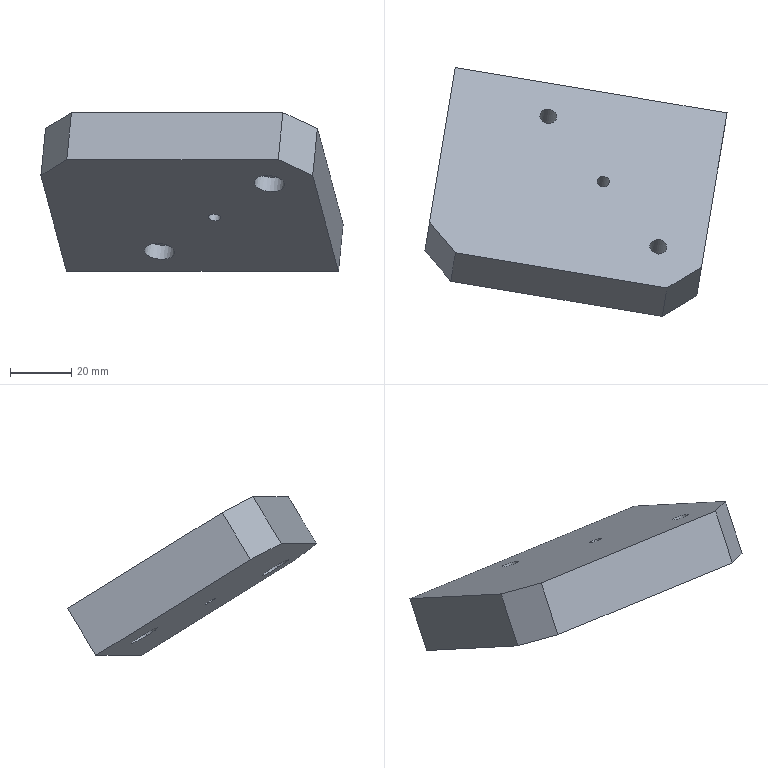Component | SolidWorks | 14AC-24-1-007-1 | 1 solid | 28 faces | box 98.73 x 81.3 x 51.9 mm | volume 109240 mm3 | cylinder 14 | plane 10 | cone 4 | commonest cylinder face diameters 10 x4 5.5 x4 5 x4 4 x2
build123d program:
from build123d import *

# Parameters (mm, degrees)
SKETCH1_W                                       = 90
SKETCH1_H                                       = 70
BOSS_EXTRUDE1_DEPTH                             = 18
CHAMFER1_SIZE                                   = 10
LPATTERN1_COUNT                                 = 2
LPATTERN1_PITCH                                 = 33
M5_HEX_SOCKET_HEAD_CAP_SCREW_CBORE1_D           = 5.5
M5_HEX_SOCKET_HEAD_CAP_SCREW_CBORE1_CBORE_D     = 10
M5_HEX_SOCKET_HEAD_CAP_SCREW_CBORE1_CBORE_DEPTH = 5.4
SKETCH12_R                                      = 2
CUT_EXTRUDE6_DEPTH                              = 116.43


with BuildPart() as part:
    # Sketch1 → Boss-Extrude1 (new body)
    with BuildSketch(Plane.XY):
        with Locations((45, 35)):
            Rectangle(SKETCH1_W, SKETCH1_H)
    extrude(amount=BOSS_EXTRUDE1_DEPTH)

    # Chamfer1
    chamfer1_edges = [part.edges().sort_by_distance(p)[0] for p in [
        (0, 70, 9),
        (90, 70, 9),
    ]]
    chamfer(chamfer1_edges, length=CHAMFER1_SIZE)

    # Sketch8 → M6 Tapped Hole1 (revolve, cut)
    with BuildSketch(Plane(origin=(18, 0, 9), x_dir=(0, 0, -1), z_dir=(1, 0, 0))):
        Polygon((0, 0), (0, 18.502), (2.5, 17), (2.5, 0), align=None)
    m6_tapped_hole1 = revolve(axis=Axis((18, -6.35, 9), (0, 1, 0)), mode=Mode.SUBTRACT)

    # LPattern1: M6 Tapped Hole1 ×2
    with Locations(*[(i * LPATTERN1_PITCH, 0, 0) for i in range(1, LPATTERN1_COUNT)]):
        add(m6_tapped_hole1, mode=Mode.SUBTRACT)

    # M5 Hex Socket Head Cap Screw CBORE1 (through all)
    with Locations(Plane(origin=(15, 55, 0), x_dir=(-1, 0, 0), z_dir=(0, 0, -1))):
        with Locations((0, 0), (-42.426, -42.426)):
            CounterBoreHole(M5_HEX_SOCKET_HEAD_CAP_SCREW_CBORE1_D / 2, M5_HEX_SOCKET_HEAD_CAP_SCREW_CBORE1_CBORE_D / 2, M5_HEX_SOCKET_HEAD_CAP_SCREW_CBORE1_CBORE_DEPTH)

    # Sketch12 → Cut-Extrude6 (cut, through all)
    with BuildSketch(Plane(origin=(0, 0, 0), x_dir=(-1, 0, 0), z_dir=(0, 0, -1))):
        with Locations((-36.213, 33.787)):
            Circle(SKETCH12_R)
    extrude(amount=-CUT_EXTRUDE6_DEPTH, mode=Mode.SUBTRACT)


solid = part.part

# Placed as in the assembly
solid = solid.moved(Location((507.217, -245.357, -123.864), (-31.129, 4.92, 171.918)))
STEP:
#1=CARTESIAN_POINT('',(18.36,-10.167,-3.578));
#2=VERTEX_POINT('',#1);
#3=CARTESIAN_POINT('',(18.515,-10.193,-3.578));
#4=VERTEX_POINT('',#3);
#5=CARTESIAN_POINT('',(18.437,-10.18,-3.578));
#6=DIRECTION('',(-0.08576,-0.5151,-0.8529));
#7=DIRECTION('',(0.9864,-0.1642,0.));
#8=AXIS2_PLACEMENT_3D('',#5,#6,#7);
#9=CIRCLE('',#8,0.07874);
#10=EDGE_CURVE('',#2,#4,#9,.T.);
#11=ORIENTED_EDGE('',*,*,#10,.F.);
#12=CARTESIAN_POINT('',(18.299,-10.532,-4.182));
#13=VERTEX_POINT('',#12);
#14=CARTESIAN_POINT('',(18.36,-10.167,-3.578));
#15=DIRECTION('',(-0.08576,-0.5151,-0.8529));
#16=VECTOR('',#15,39.37);
#17=LINE('',#14,#16);
#18=EDGE_CURVE('',#2,#13,#17,.T.);
#19=ORIENTED_EDGE('',*,*,#18,.T.);
#20=CARTESIAN_POINT('',(18.454,-10.558,-4.182));
#21=VERTEX_POINT('',#20);
#22=CARTESIAN_POINT('',(18.376,-10.545,-4.182));
#23=DIRECTION('',(-0.08576,-0.5151,-0.8529));
#24=DIRECTION('',(0.9864,-0.1642,0.));
#25=AXIS2_PLACEMENT_3D('',#22,#23,#24);
#26=CIRCLE('',#25,0.07874);
#27=EDGE_CURVE('',#13,#21,#26,.T.);
#28=ORIENTED_EDGE('',*,*,#27,.T.);
#29=CARTESIAN_POINT('',(18.515,-10.193,-3.578));
#30=DIRECTION('',(-0.08576,-0.5151,-0.8529));
#31=VECTOR('',#30,39.37);
#32=LINE('',#29,#31);
#33=EDGE_CURVE('',#4,#21,#32,.T.);
#34=ORIENTED_EDGE('',*,*,#33,.F.);
#35=EDGE_LOOP('',(#11,#19,#28,#34));
#36=FACE_OUTER_BOUND('',#35,.T.);
#37=CARTESIAN_POINT('',(18.437,-10.18,-3.578));
#38=DIRECTION('',(-0.08576,-0.5151,-0.8529));
#39=DIRECTION('',(0.9864,-0.1642,0.));
#40=AXIS2_PLACEMENT_3D('',#37,#38,#39);
#41=CYLINDRICAL_SURFACE('',#40,0.07874);
#42=ADVANCED_FACE('',(#36),#41,.F.);
#43=CARTESIAN_POINT('',(18.907,-11.243,-3.565));
#44=VERTEX_POINT('',#43);
#45=CARTESIAN_POINT('',(19.296,-11.307,-3.565));
#46=VERTEX_POINT('',#45);
#47=CARTESIAN_POINT('',(19.102,-11.275,-3.565));
#48=DIRECTION('',(-0.08576,-0.5151,-0.8529));
#49=DIRECTION('',(0.9864,-0.1642,0.));
#50=AXIS2_PLACEMENT_3D('',#47,#48,#49);
#51=CIRCLE('',#50,0.1969);
#52=EDGE_CURVE('',#44,#46,#51,.T.);
#53=ORIENTED_EDGE('',*,*,#52,.F.);
#54=CARTESIAN_POINT('',(18.889,-11.352,-3.746));
#55=VERTEX_POINT('',#54);
#56=CARTESIAN_POINT('',(18.889,-11.352,-3.746));
#57=DIRECTION('',(-0.08576,-0.5151,-0.8529));
#58=VECTOR('',#57,39.37);
#59=LINE('',#56,#58);
#60=EDGE_CURVE('',#44,#55,#59,.T.);
#61=ORIENTED_EDGE('',*,*,#60,.T.);
#62=CARTESIAN_POINT('',(19.277,-11.417,-3.746));
#63=VERTEX_POINT('',#62);
#64=CARTESIAN_POINT('',(19.083,-11.384,-3.746));
#65=DIRECTION('',(-0.08576,-0.5151,-0.8529));
#66=DIRECTION('',(0.9864,-0.1642,0.));
#67=AXIS2_PLACEMENT_3D('',#64,#65,#66);
#68=CIRCLE('',#67,0.1969);
#69=EDGE_CURVE('',#55,#63,#68,.T.);
#70=ORIENTED_EDGE('',*,*,#69,.T.);
#71=CARTESIAN_POINT('',(19.277,-11.417,-3.746));
#72=DIRECTION('',(-0.08576,-0.5151,-0.8529));
#73=VECTOR('',#72,39.37);
#74=LINE('',#71,#73);
#75=EDGE_CURVE('',#46,#63,#74,.T.);
#76=ORIENTED_EDGE('',*,*,#75,.F.);
#77=EDGE_LOOP('',(#53,#61,#70,#76));
#78=FACE_OUTER_BOUND('',#77,.T.);
#79=CARTESIAN_POINT('',(19.083,-11.384,-3.746));
#80=DIRECTION('',(-0.08576,-0.5151,-0.8529));
#81=DIRECTION('',(0.9864,-0.1642,0.));
#82=AXIS2_PLACEMENT_3D('',#79,#80,#81);
#83=CYLINDRICAL_SURFACE('',#82,0.1969);
#84=ADVANCED_FACE('',(#78),#83,.F.);
#85=CARTESIAN_POINT('',(19.037,-11.002,-3.142));
#86=VERTEX_POINT('',#85);
#87=CARTESIAN_POINT('',(19.251,-11.037,-3.142));
#88=VERTEX_POINT('',#87);
#89=CARTESIAN_POINT('',(19.144,-11.019,-3.142));
#90=DIRECTION('',(-0.08576,-0.5151,-0.8529));
#91=DIRECTION('',(0.9864,-0.1642,0.));
#92=AXIS2_PLACEMENT_3D('',#89,#90,#91);
#93=CIRCLE('',#92,0.1083);
#94=EDGE_CURVE('',#86,#88,#93,.T.);
#95=ORIENTED_EDGE('',*,*,#94,.F.);
#96=CARTESIAN_POINT('',(18.995,-11.257,-3.565));
#97=VERTEX_POINT('',#96);
#98=CARTESIAN_POINT('',(18.977,-11.367,-3.746));
#99=DIRECTION('',(-0.08576,-0.5151,-0.8529));
#100=VECTOR('',#99,39.37);
#101=LINE('',#98,#100);
#102=EDGE_CURVE('',#86,#97,#101,.T.);
#103=ORIENTED_EDGE('',*,*,#102,.T.);
#104=CARTESIAN_POINT('',(19.208,-11.293,-3.565));
#105=VERTEX_POINT('',#104);
#106=CARTESIAN_POINT('',(19.102,-11.275,-3.565));
#107=DIRECTION('',(-0.08576,-0.5151,-0.8529));
#108=DIRECTION('',(0.9864,-0.1642,0.));
#109=AXIS2_PLACEMENT_3D('',#106,#107,#108);
#110=CIRCLE('',#109,0.1083);
#111=EDGE_CURVE('',#97,#105,#110,.T.);
#112=ORIENTED_EDGE('',*,*,#111,.T.);
#113=CARTESIAN_POINT('',(19.19,-11.402,-3.746));
#114=DIRECTION('',(-0.08576,-0.5151,-0.8529));
#115=VECTOR('',#114,39.37);
#116=LINE('',#113,#115);
#117=EDGE_CURVE('',#88,#105,#116,.T.);
#118=ORIENTED_EDGE('',*,*,#117,.F.);
#119=EDGE_LOOP('',(#95,#103,#112,#118));
#120=FACE_OUTER_BOUND('',#119,.T.);
#121=CARTESIAN_POINT('',(19.083,-11.384,-3.746));
#122=DIRECTION('',(-0.08576,-0.5151,-0.8529));
#123=DIRECTION('',(0.9864,-0.1642,0.));
#124=AXIS2_PLACEMENT_3D('',#121,#122,#123);
#125=CYLINDRICAL_SURFACE('',#124,0.1083);
#126=ADVANCED_FACE('',(#120),#125,.F.);
#127=CARTESIAN_POINT('',(17.494,-9.563,-4.437));
#128=VERTEX_POINT('',#127);
#129=CARTESIAN_POINT('',(17.882,-9.628,-4.437));
#130=VERTEX_POINT('',#129);
#131=CARTESIAN_POINT('',(17.688,-9.595,-4.437));
#132=DIRECTION('',(-0.08576,-0.5151,-0.8529));
#133=DIRECTION('',(0.9864,-0.1642,0.));
#134=AXIS2_PLACEMENT_3D('',#131,#132,#133);
#135=CIRCLE('',#134,0.1969);
#136=EDGE_CURVE('',#128,#130,#135,.T.);
#137=ORIENTED_EDGE('',*,*,#136,.F.);
#138=CARTESIAN_POINT('',(17.475,-9.673,-4.618));
#139=VERTEX_POINT('',#138);
#140=CARTESIAN_POINT('',(17.475,-9.673,-4.618));
#141=DIRECTION('',(-0.08576,-0.5151,-0.8529));
#142=VECTOR('',#141,39.37);
#143=LINE('',#140,#142);
#144=EDGE_CURVE('',#128,#139,#143,.T.);
#145=ORIENTED_EDGE('',*,*,#144,.T.);
#146=CARTESIAN_POINT('',(17.864,-9.737,-4.618));
#147=VERTEX_POINT('',#146);
#148=CARTESIAN_POINT('',(17.67,-9.705,-4.618));
#149=DIRECTION('',(-0.08576,-0.5151,-0.8529));
#150=DIRECTION('',(0.9864,-0.1642,0.));
#151=AXIS2_PLACEMENT_3D('',#148,#149,#150);
#152=CIRCLE('',#151,0.1969);
#153=EDGE_CURVE('',#139,#147,#152,.T.);
#154=ORIENTED_EDGE('',*,*,#153,.T.);
#155=CARTESIAN_POINT('',(17.864,-9.737,-4.618));
#156=DIRECTION('',(-0.08576,-0.5151,-0.8529));
#157=VECTOR('',#156,39.37);
#158=LINE('',#155,#157);
#159=EDGE_CURVE('',#130,#147,#158,.T.);
#160=ORIENTED_EDGE('',*,*,#159,.F.);
#161=EDGE_LOOP('',(#137,#145,#154,#160));
#162=FACE_OUTER_BOUND('',#161,.T.);
#163=CARTESIAN_POINT('',(17.67,-9.705,-4.618));
#164=DIRECTION('',(-0.08576,-0.5151,-0.8529));
#165=DIRECTION('',(0.9864,-0.1642,0.));
#166=AXIS2_PLACEMENT_3D('',#163,#164,#165);
#167=CYLINDRICAL_SURFACE('',#166,0.1969);
#168=ADVANCED_FACE('',(#162),#167,.F.);
#169=CARTESIAN_POINT('',(17.624,-9.322,-4.014));
#170=VERTEX_POINT('',#169);
#171=CARTESIAN_POINT('',(17.837,-9.358,-4.014));
#172=VERTEX_POINT('',#171);
#173=CARTESIAN_POINT('',(17.73,-9.34,-4.014));
#174=DIRECTION('',(-0.08576,-0.5151,-0.8529));
#175=DIRECTION('',(0.9864,-0.1642,0.));
#176=AXIS2_PLACEMENT_3D('',#173,#174,#175);
#177=CIRCLE('',#176,0.1083);
#178=EDGE_CURVE('',#170,#172,#177,.T.);
#179=ORIENTED_EDGE('',*,*,#178,.F.);
#180=CARTESIAN_POINT('',(17.581,-9.578,-4.437));
#181=VERTEX_POINT('',#180);
#182=CARTESIAN_POINT('',(17.563,-9.687,-4.618));
#183=DIRECTION('',(-0.08576,-0.5151,-0.8529));
#184=VECTOR('',#183,39.37);
#185=LINE('',#182,#184);
#186=EDGE_CURVE('',#170,#181,#185,.T.);
#187=ORIENTED_EDGE('',*,*,#186,.T.);
#188=CARTESIAN_POINT('',(17.795,-9.613,-4.437));
#189=VERTEX_POINT('',#188);
#190=CARTESIAN_POINT('',(17.688,-9.595,-4.437));
#191=DIRECTION('',(-0.08576,-0.5151,-0.8529));
#192=DIRECTION('',(0.9864,-0.1642,0.));
#193=AXIS2_PLACEMENT_3D('',#190,#191,#192);
#194=CIRCLE('',#193,0.1083);
#195=EDGE_CURVE('',#181,#189,#194,.T.);
#196=ORIENTED_EDGE('',*,*,#195,.T.);
#197=CARTESIAN_POINT('',(17.776,-9.723,-4.618));
#198=DIRECTION('',(-0.08576,-0.5151,-0.8529));
#199=VECTOR('',#198,39.37);
#200=LINE('',#197,#199);
#201=EDGE_CURVE('',#172,#189,#200,.T.);
#202=ORIENTED_EDGE('',*,*,#201,.F.);
#203=EDGE_LOOP('',(#179,#187,#196,#202));
#204=FACE_OUTER_BOUND('',#203,.T.);
#205=CARTESIAN_POINT('',(17.67,-9.705,-4.618));
#206=DIRECTION('',(-0.08576,-0.5151,-0.8529));
#207=DIRECTION('',(0.9864,-0.1642,0.));
#208=AXIS2_PLACEMENT_3D('',#205,#206,#207);
#209=CYLINDRICAL_SURFACE('',#208,0.1083);
#210=ADVANCED_FACE('',(#204),#209,.F.);
#211=CARTESIAN_POINT('',(17.934,-9.66,-4.141));
#212=VERTEX_POINT('',#211);
#213=CARTESIAN_POINT('',(17.917,-9.761,-4.309));
#214=VERTEX_POINT('',#213);
#215=CARTESIAN_POINT('',(17.925,-9.711,-4.225));
#216=DIRECTION('',(0.1401,0.8413,-0.5222));
#217=DIRECTION('',(-0.08576,-0.5151,-0.8529));
#218=AXIS2_PLACEMENT_3D('',#215,#216,#217);
#219=CIRCLE('',#218,0.09843);
#220=EDGE_CURVE('',#212,#214,#219,.T.);
#221=ORIENTED_EDGE('',*,*,#220,.F.);
#222=CARTESIAN_POINT('',(18.027,-9.097,-4.49));
#223=VERTEX_POINT('',#222);
#224=CARTESIAN_POINT('',(18.027,-9.097,-4.49));
#225=DIRECTION('',(0.1401,0.8413,-0.5222));
#226=VECTOR('',#225,39.37);
#227=LINE('',#224,#226);
#228=EDGE_CURVE('',#212,#223,#227,.T.);
#229=ORIENTED_EDGE('',*,*,#228,.T.);
#230=CARTESIAN_POINT('',(18.01,-9.198,-4.658));
#231=VERTEX_POINT('',#230);
#232=CARTESIAN_POINT('',(18.019,-9.147,-4.574));
#233=DIRECTION('',(0.1401,0.8413,-0.5222));
#234=DIRECTION('',(-0.08576,-0.5151,-0.8529));
#235=AXIS2_PLACEMENT_3D('',#232,#233,#234);
#236=CIRCLE('',#235,0.09843);
#237=EDGE_CURVE('',#223,#231,#236,.T.);
#238=ORIENTED_EDGE('',*,*,#237,.T.);
#239=CARTESIAN_POINT('',(18.01,-9.198,-4.658));
#240=DIRECTION('',(0.1401,0.8413,-0.5222));
#241=VECTOR('',#240,39.37);
#242=LINE('',#239,#241);
#243=EDGE_CURVE('',#214,#231,#242,.T.);
#244=ORIENTED_EDGE('',*,*,#243,.F.);
#245=EDGE_LOOP('',(#221,#229,#238,#244));
#246=FACE_OUTER_BOUND('',#245,.T.);
#247=CARTESIAN_POINT('',(18.019,-9.147,-4.574));
#248=DIRECTION('',(0.1401,0.8413,-0.5222));
#249=DIRECTION('',(-0.08576,-0.5151,-0.8529));
#250=AXIS2_PLACEMENT_3D('',#247,#248,#249);
#251=CYLINDRICAL_SURFACE('',#250,0.09843);
#252=ADVANCED_FACE('',(#246),#251,.F.);
#253=CARTESIAN_POINT('',(17.917,-9.76,-4.194));
#254=VERTEX_POINT('',#253);
#255=CARTESIAN_POINT('',(17.917,-9.761,-4.309));
#256=DIRECTION('',(-0.001367,-0.008211,-1.));
#257=VECTOR('',#256,39.37);
#258=LINE('',#255,#257);
#259=EDGE_CURVE('',#254,#214,#258,.T.);
#260=ORIENTED_EDGE('',*,*,#259,.F.);
#261=CARTESIAN_POINT('',(17.934,-9.66,-4.141));
#262=DIRECTION('',(0.1457,0.8748,0.4621));
#263=VECTOR('',#262,39.37);
#264=LINE('',#261,#263);
#265=EDGE_CURVE('',#254,#212,#264,.T.);
#266=ORIENTED_EDGE('',*,*,#265,.T.);
#267=ORIENTED_EDGE('',*,*,#220,.T.);
#268=EDGE_LOOP('',(#260,#266,#267));
#269=FACE_OUTER_BOUND('',#268,.T.);
#270=CARTESIAN_POINT('',(17.925,-9.711,-4.225));
#271=DIRECTION('',(0.1401,0.8413,-0.5222));
#272=DIRECTION('',(-0.08576,-0.5151,-0.8529));
#273=AXIS2_PLACEMENT_3D('',#270,#271,#272);
#274=CONICAL_SURFACE('',#273,0.09843,1.03);
#275=ADVANCED_FACE('',(#269),#274,.F.);
#276=CARTESIAN_POINT('',(19.215,-9.873,-4.141));
#277=VERTEX_POINT('',#276);
#278=CARTESIAN_POINT('',(19.198,-9.975,-4.309));
#279=VERTEX_POINT('',#278);
#280=CARTESIAN_POINT('',(19.207,-9.924,-4.225));
#281=DIRECTION('',(0.1401,0.8413,-0.5222));
#282=DIRECTION('',(-0.08576,-0.5151,-0.8529));
#283=AXIS2_PLACEMENT_3D('',#280,#281,#282);
#284=CIRCLE('',#283,0.09843);
#285=EDGE_CURVE('',#277,#279,#284,.T.);
#286=ORIENTED_EDGE('',*,*,#285,.F.);
#287=CARTESIAN_POINT('',(19.309,-9.31,-4.49));
#288=VERTEX_POINT('',#287);
#289=CARTESIAN_POINT('',(19.309,-9.31,-4.49));
#290=DIRECTION('',(0.1401,0.8413,-0.5222));
#291=VECTOR('',#290,39.37);
#292=LINE('',#289,#291);
#293=EDGE_CURVE('',#277,#288,#292,.T.);
#294=ORIENTED_EDGE('',*,*,#293,.T.);
#295=CARTESIAN_POINT('',(19.292,-9.412,-4.658));
#296=VERTEX_POINT('',#295);
#297=CARTESIAN_POINT('',(19.301,-9.361,-4.574));
#298=DIRECTION('',(0.1401,0.8413,-0.5222));
#299=DIRECTION('',(-0.08576,-0.5151,-0.8529));
#300=AXIS2_PLACEMENT_3D('',#297,#298,#299);
#301=CIRCLE('',#300,0.09843);
#302=EDGE_CURVE('',#288,#296,#301,.T.);
#303=ORIENTED_EDGE('',*,*,#302,.T.);
#304=CARTESIAN_POINT('',(19.292,-9.412,-4.658));
#305=DIRECTION('',(0.1401,0.8413,-0.5222));
#306=VECTOR('',#305,39.37);
#307=LINE('',#304,#306);
#308=EDGE_CURVE('',#279,#296,#307,.T.);
#309=ORIENTED_EDGE('',*,*,#308,.F.);
#310=EDGE_LOOP('',(#286,#294,#303,#309));
#311=FACE_OUTER_BOUND('',#310,.T.);
#312=CARTESIAN_POINT('',(19.301,-9.361,-4.574));
#313=DIRECTION('',(0.1401,0.8413,-0.5222));
#314=DIRECTION('',(-0.08576,-0.5151,-0.8529));
#315=AXIS2_PLACEMENT_3D('',#312,#313,#314);
#316=CYLINDRICAL_SURFACE('',#315,0.09843);
#317=ADVANCED_FACE('',(#311),#316,.F.);
#318=CARTESIAN_POINT('',(19.198,-9.974,-4.194));
#319=VERTEX_POINT('',#318);
#320=CARTESIAN_POINT('',(19.198,-9.975,-4.309));
#321=DIRECTION('',(-0.001367,-0.008211,-1.));
#322=VECTOR('',#321,39.37);
#323=LINE('',#320,#322);
#324=EDGE_CURVE('',#319,#279,#323,.T.);
#325=ORIENTED_EDGE('',*,*,#324,.F.);
#326=CARTESIAN_POINT('',(19.215,-9.873,-4.141));
#327=DIRECTION('',(0.1457,0.8748,0.4621));
#328=VECTOR('',#327,39.37);
#329=LINE('',#326,#328);
#330=EDGE_CURVE('',#319,#277,#329,.T.);
#331=ORIENTED_EDGE('',*,*,#330,.T.);
#332=ORIENTED_EDGE('',*,*,#285,.T.);
#333=EDGE_LOOP('',(#325,#331,#332));
#334=FACE_OUTER_BOUND('',#333,.T.);
#335=CARTESIAN_POINT('',(19.207,-9.924,-4.225));
#336=DIRECTION('',(0.1401,0.8413,-0.5222));
#337=DIRECTION('',(-0.08576,-0.5151,-0.8529));
#338=AXIS2_PLACEMENT_3D('',#335,#336,#337);
#339=CONICAL_SURFACE('',#338,0.09843,1.03);
#340=ADVANCED_FACE('',(#334),#339,.F.);
#341=CARTESIAN_POINT('',(19.699,-11.282,-3.039));
#342=VERTEX_POINT('',#341);
#343=CARTESIAN_POINT('',(20.03,-9.295,-4.272));
#344=VERTEX_POINT('',#343);
#345=CARTESIAN_POINT('',(20.03,-9.295,-4.272));
#346=DIRECTION('',(0.1401,0.8413,-0.5222));
#347=VECTOR('',#346,39.37);
#348=LINE('',#345,#347);
#349=EDGE_CURVE('',#342,#344,#348,.T.);
#350=ORIENTED_EDGE('',*,*,#349,.F.);
#351=CARTESIAN_POINT('',(19.638,-11.647,-3.643));
#352=VERTEX_POINT('',#351);
#353=CARTESIAN_POINT('',(19.699,-11.282,-3.039));
#354=DIRECTION('',(-0.08576,-0.5151,-0.8529));
#355=VECTOR('',#354,39.37);
#356=LINE('',#353,#355);
#357=EDGE_CURVE('',#342,#352,#356,.T.);
#358=ORIENTED_EDGE('',*,*,#357,.T.);
#359=CARTESIAN_POINT('',(19.969,-9.66,-4.877));
#360=VERTEX_POINT('',#359);
#361=CARTESIAN_POINT('',(19.969,-9.66,-4.877));
#362=DIRECTION('',(0.1401,0.8413,-0.5222));
#363=VECTOR('',#362,39.37);
#364=LINE('',#361,#363);
#365=EDGE_CURVE('',#352,#360,#364,.T.);
#366=ORIENTED_EDGE('',*,*,#365,.T.);
#367=CARTESIAN_POINT('',(20.03,-9.295,-4.272));
#368=DIRECTION('',(-0.08576,-0.5151,-0.8529));
#369=VECTOR('',#368,39.37);
#370=LINE('',#367,#369);
#371=EDGE_CURVE('',#344,#360,#370,.T.);
#372=ORIENTED_EDGE('',*,*,#371,.F.);
#373=EDGE_LOOP('',(#350,#358,#366,#372));
#374=FACE_OUTER_BOUND('',#373,.T.);
#375=CARTESIAN_POINT('',(20.03,-9.295,-4.272));
#376=DIRECTION('',(-0.9864,0.1642,0.));
#377=DIRECTION('',(-0.08576,-0.5151,-0.8529));
#378=AXIS2_PLACEMENT_3D('',#375,#376,#377);
#379=PLANE('',#378);
#380=ADVANCED_FACE('',(#374),#379,.F.);
#381=CARTESIAN_POINT('',(18.019,-9.147,-4.574));
#382=DIRECTION('',(0.1401,0.8413,-0.5222));
#383=DIRECTION('',(-0.08576,-0.5151,-0.8529));
#384=AXIS2_PLACEMENT_3D('',#381,#382,#383);
#385=CIRCLE('',#384,0.09843);
#386=EDGE_CURVE('',#231,#223,#385,.T.);
#387=ORIENTED_EDGE('',*,*,#386,.F.);
#388=ORIENTED_EDGE('',*,*,#237,.F.);
#389=EDGE_LOOP('',(#387,#388));
#390=FACE_BOUND('',#389,.T.);
#391=CARTESIAN_POINT('',(19.301,-9.361,-4.574));
#392=DIRECTION('',(0.1401,0.8413,-0.5222));
#393=DIRECTION('',(-0.08576,-0.5151,-0.8529));
#394=AXIS2_PLACEMENT_3D('',#391,#392,#393);
#395=CIRCLE('',#394,0.09843);
#396=EDGE_CURVE('',#296,#288,#395,.T.);
#397=ORIENTED_EDGE('',*,*,#396,.F.);
#398=ORIENTED_EDGE('',*,*,#302,.F.);
#399=EDGE_LOOP('',(#397,#398));
#400=FACE_BOUND('',#399,.T.);
#401=CARTESIAN_POINT('',(16.474,-9.078,-4.877));
#402=VERTEX_POINT('',#401);
#403=CARTESIAN_POINT('',(19.969,-9.66,-4.877));
#404=DIRECTION('',(-0.9864,0.1642,0.));
#405=VECTOR('',#404,39.37);
#406=LINE('',#403,#405);
#407=EDGE_CURVE('',#360,#402,#406,.T.);
#408=ORIENTED_EDGE('',*,*,#407,.T.);
#409=CARTESIAN_POINT('',(16.535,-8.713,-4.272));
#410=VERTEX_POINT('',#409);
#411=CARTESIAN_POINT('',(16.535,-8.713,-4.272));
#412=DIRECTION('',(-0.08576,-0.5151,-0.8529));
#413=VECTOR('',#412,39.37);
#414=LINE('',#411,#413);
#415=EDGE_CURVE('',#410,#402,#414,.T.);
#416=ORIENTED_EDGE('',*,*,#415,.F.);
#417=CARTESIAN_POINT('',(20.03,-9.295,-4.272));
#418=DIRECTION('',(-0.9864,0.1642,0.));
#419=VECTOR('',#418,39.37);
#420=LINE('',#417,#419);
#421=EDGE_CURVE('',#344,#410,#420,.T.);
#422=ORIENTED_EDGE('',*,*,#421,.F.);
#423=ORIENTED_EDGE('',*,*,#371,.T.);
#424=EDGE_LOOP('',(#408,#416,#422,#423));
#425=FACE_OUTER_BOUND('',#424,.T.);
#426=CARTESIAN_POINT('',(20.03,-9.295,-4.272));
#427=DIRECTION('',(-0.1401,-0.8413,0.5222));
#428=DIRECTION('',(0.08576,0.5151,0.8529));
#429=AXIS2_PLACEMENT_3D('',#426,#427,#428);
#430=PLANE('',#429);
#431=ADVANCED_FACE('',(#390,#400,#425),#430,.F.);
#432=CARTESIAN_POINT('',(16.143,-11.065,-3.643));
#433=VERTEX_POINT('',#432);
#434=CARTESIAN_POINT('',(16.474,-9.078,-4.877));
#435=DIRECTION('',(-0.1401,-0.8413,0.5222));
#436=VECTOR('',#435,39.37);
#437=LINE('',#434,#436);
#438=EDGE_CURVE('',#402,#433,#437,.T.);
#439=ORIENTED_EDGE('',*,*,#438,.T.);
#440=CARTESIAN_POINT('',(16.204,-10.7,-3.039));
#441=VERTEX_POINT('',#440);
#442=CARTESIAN_POINT('',(16.204,-10.7,-3.039));
#443=DIRECTION('',(0.08576,0.5151,0.8529));
#444=VECTOR('',#443,39.37);
#445=LINE('',#442,#444);
#446=EDGE_CURVE('',#433,#441,#445,.T.);
#447=ORIENTED_EDGE('',*,*,#446,.T.);
#448=CARTESIAN_POINT('',(16.535,-8.713,-4.272));
#449=DIRECTION('',(-0.1401,-0.8413,0.5222));
#450=VECTOR('',#449,39.37);
#451=LINE('',#448,#450);
#452=EDGE_CURVE('',#410,#441,#451,.T.);
#453=ORIENTED_EDGE('',*,*,#452,.F.);
#454=ORIENTED_EDGE('',*,*,#415,.T.);
#455=EDGE_LOOP('',(#439,#447,#453,#454));
#456=FACE_OUTER_BOUND('',#455,.T.);
#457=CARTESIAN_POINT('',(16.535,-8.713,-4.272));
#458=DIRECTION('',(0.9864,-0.1642,-0.));
#459=DIRECTION('',(0.08576,0.5151,0.8529));
#460=AXIS2_PLACEMENT_3D('',#457,#458,#459);
#461=PLANE('',#460);
#462=ADVANCED_FACE('',(#456),#461,.F.);
#463=CARTESIAN_POINT('',(16.537,-11.096,-2.833));
#464=VERTEX_POINT('',#463);
#465=CARTESIAN_POINT('',(19.256,-11.549,-2.833));
#466=VERTEX_POINT('',#465);
#467=CARTESIAN_POINT('',(19.644,-11.613,-2.833));
#468=DIRECTION('',(0.9864,-0.1642,-0.));
#469=VECTOR('',#468,39.37);
#470=LINE('',#467,#469);
#471=EDGE_CURVE('',#464,#466,#470,.T.);
#472=ORIENTED_EDGE('',*,*,#471,.F.);
#473=CARTESIAN_POINT('',(16.476,-11.461,-3.438));
#474=VERTEX_POINT('',#473);
#475=CARTESIAN_POINT('',(16.537,-11.096,-2.833));
#476=DIRECTION('',(-0.08576,-0.5151,-0.8529));
#477=VECTOR('',#476,39.37);
#478=LINE('',#475,#477);
#479=EDGE_CURVE('',#464,#474,#478,.T.);
#480=ORIENTED_EDGE('',*,*,#479,.T.);
#481=CARTESIAN_POINT('',(19.195,-11.914,-3.438));
#482=VERTEX_POINT('',#481);
#483=CARTESIAN_POINT('',(19.583,-11.978,-3.438));
#484=DIRECTION('',(0.9864,-0.1642,-0.));
#485=VECTOR('',#484,39.37);
#486=LINE('',#483,#485);
#487=EDGE_CURVE('',#474,#482,#486,.T.);
#488=ORIENTED_EDGE('',*,*,#487,.T.);
#489=CARTESIAN_POINT('',(19.256,-11.549,-2.833));
#490=DIRECTION('',(0.08576,0.5151,0.8529));
#491=VECTOR('',#490,39.37);
#492=LINE('',#489,#491);
#493=EDGE_CURVE('',#482,#466,#492,.T.);
#494=ORIENTED_EDGE('',*,*,#493,.T.);
#495=EDGE_LOOP('',(#472,#480,#488,#494));
#496=FACE_OUTER_BOUND('',#495,.T.);
#497=CARTESIAN_POINT('',(19.644,-11.613,-2.833));
#498=DIRECTION('',(0.1401,0.8413,-0.5222));
#499=DIRECTION('',(-0.08576,-0.5151,-0.8529));
#500=AXIS2_PLACEMENT_3D('',#497,#498,#499);
#501=PLANE('',#500);
#502=ADVANCED_FACE('',(#496),#501,.F.);
#503=CARTESIAN_POINT('',(18.437,-10.18,-3.578));
#504=DIRECTION('',(-0.08576,-0.5151,-0.8529));
#505=DIRECTION('',(0.9864,-0.1642,0.));
#506=AXIS2_PLACEMENT_3D('',#503,#504,#505);
#507=CIRCLE('',#506,0.07874);
#508=EDGE_CURVE('',#4,#2,#507,.T.);
#509=ORIENTED_EDGE('',*,*,#508,.T.);
#510=ORIENTED_EDGE('',*,*,#10,.T.);
#511=EDGE_LOOP('',(#509,#510));
#512=FACE_BOUND('',#511,.T.);
#513=CARTESIAN_POINT('',(19.144,-11.019,-3.142));
#514=DIRECTION('',(-0.08576,-0.5151,-0.8529));
#515=DIRECTION('',(0.9864,-0.1642,0.));
#516=AXIS2_PLACEMENT_3D('',#513,#514,#515);
#517=CIRCLE('',#516,0.1083);
#518=EDGE_CURVE('',#88,#86,#517,.T.);
#519=ORIENTED_EDGE('',*,*,#518,.T.);
#520=ORIENTED_EDGE('',*,*,#94,.T.);
#521=EDGE_LOOP('',(#519,#520));
#522=FACE_BOUND('',#521,.T.);
#523=CARTESIAN_POINT('',(17.73,-9.34,-4.014));
#524=DIRECTION('',(-0.08576,-0.5151,-0.8529));
#525=DIRECTION('',(0.9864,-0.1642,0.));
#526=AXIS2_PLACEMENT_3D('',#523,#524,#525);
#527=CIRCLE('',#526,0.1083);
#528=EDGE_CURVE('',#172,#170,#527,.T.);
#529=ORIENTED_EDGE('',*,*,#528,.T.);
#530=ORIENTED_EDGE('',*,*,#178,.T.);
#531=EDGE_LOOP('',(#529,#530));
#532=FACE_BOUND('',#531,.T.);
#533=ORIENTED_EDGE('',*,*,#452,.T.);
#534=CARTESIAN_POINT('',(16.537,-11.096,-2.833));
#535=DIRECTION('',(0.5985,-0.711,0.3692));
#536=VECTOR('',#535,39.37);
#537=LINE('',#534,#536);
#538=EDGE_CURVE('',#441,#464,#537,.T.);
#539=ORIENTED_EDGE('',*,*,#538,.T.);
#540=ORIENTED_EDGE('',*,*,#471,.T.);
#541=CARTESIAN_POINT('',(19.699,-11.282,-3.039));
#542=DIRECTION('',(0.7966,0.4787,-0.3692));
#543=VECTOR('',#542,39.37);
#544=LINE('',#541,#543);
#545=EDGE_CURVE('',#466,#342,#544,.T.);
#546=ORIENTED_EDGE('',*,*,#545,.T.);
#547=ORIENTED_EDGE('',*,*,#349,.T.);
#548=ORIENTED_EDGE('',*,*,#421,.T.);
#549=EDGE_LOOP('',(#533,#539,#540,#546,#547,#548));
#550=FACE_OUTER_BOUND('',#549,.T.);
#551=CARTESIAN_POINT('',(19.644,-11.613,-2.833));
#552=DIRECTION('',(-0.08576,-0.5151,-0.8529));
#553=DIRECTION('',(0.9864,-0.1642,-0.));
#554=AXIS2_PLACEMENT_3D('',#551,#552,#553);
#555=PLANE('',#554);
#556=ADVANCED_FACE('',(#512,#522,#532,#550),#555,.F.);
#557=CARTESIAN_POINT('',(18.376,-10.545,-4.182));
#558=DIRECTION('',(-0.08576,-0.5151,-0.8529));
#559=DIRECTION('',(0.9864,-0.1642,0.));
#560=AXIS2_PLACEMENT_3D('',#557,#558,#559);
#561=CIRCLE('',#560,0.07874);
#562=EDGE_CURVE('',#21,#13,#561,.T.);
#563=ORIENTED_EDGE('',*,*,#562,.F.);
#564=ORIENTED_EDGE('',*,*,#27,.F.);
#565=EDGE_LOOP('',(#563,#564));
#566=FACE_BOUND('',#565,.T.);
#567=CARTESIAN_POINT('',(19.083,-11.384,-3.746));
#568=DIRECTION('',(-0.08576,-0.5151,-0.8529));
#569=DIRECTION('',(0.9864,-0.1642,0.));
#570=AXIS2_PLACEMENT_3D('',#567,#568,#569);
#571=CIRCLE('',#570,0.1969);
#572=EDGE_CURVE('',#63,#55,#571,.T.);
#573=ORIENTED_EDGE('',*,*,#572,.F.);
#574=ORIENTED_EDGE('',*,*,#69,.F.);
#575=EDGE_LOOP('',(#573,#574));
#576=FACE_BOUND('',#575,.T.);
#577=CARTESIAN_POINT('',(17.67,-9.705,-4.618));
#578=DIRECTION('',(-0.08576,-0.5151,-0.8529));
#579=DIRECTION('',(0.9864,-0.1642,0.));
#580=AXIS2_PLACEMENT_3D('',#577,#578,#579);
#581=CIRCLE('',#580,0.1969);
#582=EDGE_CURVE('',#147,#139,#581,.T.);
#583=ORIENTED_EDGE('',*,*,#582,.F.);
#584=ORIENTED_EDGE('',*,*,#153,.F.);
#585=EDGE_LOOP('',(#583,#584));
#586=FACE_BOUND('',#585,.T.);
#587=ORIENTED_EDGE('',*,*,#487,.F.);
#588=CARTESIAN_POINT('',(17.809,-13.044,-2.615));
#589=DIRECTION('',(-0.5985,0.711,-0.3692));
#590=VECTOR('',#589,39.37);
#591=LINE('',#588,#590);
#592=EDGE_CURVE('',#474,#433,#591,.T.);
#593=ORIENTED_EDGE('',*,*,#592,.T.);
#594=ORIENTED_EDGE('',*,*,#438,.F.);
#595=ORIENTED_EDGE('',*,*,#407,.F.);
#596=ORIENTED_EDGE('',*,*,#365,.F.);
#597=CARTESIAN_POINT('',(19.417,-11.78,-3.54));
#598=DIRECTION('',(-0.7966,-0.4787,0.3692));
#599=VECTOR('',#598,39.37);
#600=LINE('',#597,#599);
#601=EDGE_CURVE('',#352,#482,#600,.T.);
#602=ORIENTED_EDGE('',*,*,#601,.T.);
#603=EDGE_LOOP('',(#587,#593,#594,#595,#596,#602));
#604=FACE_OUTER_BOUND('',#603,.T.);
#605=CARTESIAN_POINT('',(19.583,-11.978,-3.438));
#606=DIRECTION('',(-0.08576,-0.5151,-0.8529));
#607=DIRECTION('',(0.9864,-0.1642,-0.));
#608=AXIS2_PLACEMENT_3D('',#605,#606,#607);
#609=PLANE('',#608);
#610=ADVANCED_FACE('',(#566,#576,#586,#604),#609,.T.);
#611=ORIENTED_EDGE('',*,*,#538,.F.);
#612=ORIENTED_EDGE('',*,*,#446,.F.);
#613=ORIENTED_EDGE('',*,*,#592,.F.);
#614=ORIENTED_EDGE('',*,*,#479,.F.);
#615=EDGE_LOOP('',(#611,#612,#613,#614));
#616=FACE_OUTER_BOUND('',#615,.T.);
#617=CARTESIAN_POINT('',(16.537,-11.096,-2.833));
#618=DIRECTION('',(0.7966,0.4787,-0.3692));
#619=DIRECTION('',(-0.5985,0.711,-0.3692));
#620=AXIS2_PLACEMENT_3D('',#617,#618,#619);
#621=PLANE('',#620);
#622=ADVANCED_FACE('',(#616),#621,.F.);
#623=ORIENTED_EDGE('',*,*,#545,.F.);
#624=ORIENTED_EDGE('',*,*,#493,.F.);
#625=ORIENTED_EDGE('',*,*,#601,.F.);
#626=ORIENTED_EDGE('',*,*,#357,.F.);
#627=EDGE_LOOP('',(#623,#624,#625,#626));
#628=FACE_OUTER_BOUND('',#627,.T.);
#629=CARTESIAN_POINT('',(19.699,-11.282,-3.039));
#630=DIRECTION('',(-0.5985,0.711,-0.3692));
#631=DIRECTION('',(-0.7966,-0.4787,0.3692));
#632=AXIS2_PLACEMENT_3D('',#629,#630,#631);
#633=PLANE('',#632);
#634=ADVANCED_FACE('',(#628),#633,.F.);
#635=ORIENTED_EDGE('',*,*,#330,.F.);
#636=ORIENTED_EDGE('',*,*,#324,.T.);
#637=CARTESIAN_POINT('',(19.207,-9.924,-4.225));
#638=DIRECTION('',(0.1401,0.8413,-0.5222));
#639=DIRECTION('',(-0.08576,-0.5151,-0.8529));
#640=AXIS2_PLACEMENT_3D('',#637,#638,#639);
#641=CIRCLE('',#640,0.09843);
#642=EDGE_CURVE('',#279,#277,#641,.T.);
#643=ORIENTED_EDGE('',*,*,#642,.T.);
#644=EDGE_LOOP('',(#635,#636,#643));
#645=FACE_OUTER_BOUND('',#644,.T.);
#646=CARTESIAN_POINT('',(19.207,-9.924,-4.225));
#647=DIRECTION('',(0.1401,0.8413,-0.5222));
#648=DIRECTION('',(-0.08576,-0.5151,-0.8529));
#649=AXIS2_PLACEMENT_3D('',#646,#647,#648);
#650=CONICAL_SURFACE('',#649,0.09843,1.03);
#651=ADVANCED_FACE('',(#645),#650,.F.);
#652=ORIENTED_EDGE('',*,*,#293,.F.);
#653=ORIENTED_EDGE('',*,*,#642,.F.);
#654=ORIENTED_EDGE('',*,*,#308,.T.);
#655=ORIENTED_EDGE('',*,*,#396,.T.);
#656=EDGE_LOOP('',(#652,#653,#654,#655));
#657=FACE_OUTER_BOUND('',#656,.T.);
#658=CARTESIAN_POINT('',(19.301,-9.361,-4.574));
#659=DIRECTION('',(0.1401,0.8413,-0.5222));
#660=DIRECTION('',(-0.08576,-0.5151,-0.8529));
#661=AXIS2_PLACEMENT_3D('',#658,#659,#660);
#662=CYLINDRICAL_SURFACE('',#661,0.09843);
#663=ADVANCED_FACE('',(#657),#662,.F.);
#664=ORIENTED_EDGE('',*,*,#265,.F.);
#665=ORIENTED_EDGE('',*,*,#259,.T.);
#666=CARTESIAN_POINT('',(17.925,-9.711,-4.225));
#667=DIRECTION('',(0.1401,0.8413,-0.5222));
#668=DIRECTION('',(-0.08576,-0.5151,-0.8529));
#669=AXIS2_PLACEMENT_3D('',#666,#667,#668);
#670=CIRCLE('',#669,0.09843);
#671=EDGE_CURVE('',#214,#212,#670,.T.);
#672=ORIENTED_EDGE('',*,*,#671,.T.);
#673=EDGE_LOOP('',(#664,#665,#672));
#674=FACE_OUTER_BOUND('',#673,.T.);
#675=CARTESIAN_POINT('',(17.925,-9.711,-4.225));
#676=DIRECTION('',(0.1401,0.8413,-0.5222));
#677=DIRECTION('',(-0.08576,-0.5151,-0.8529));
#678=AXIS2_PLACEMENT_3D('',#675,#676,#677);
#679=CONICAL_SURFACE('',#678,0.09843,1.03);
#680=ADVANCED_FACE('',(#674),#679,.F.);
#681=ORIENTED_EDGE('',*,*,#228,.F.);
#682=ORIENTED_EDGE('',*,*,#671,.F.);
#683=ORIENTED_EDGE('',*,*,#243,.T.);
#684=ORIENTED_EDGE('',*,*,#386,.T.);
#685=EDGE_LOOP('',(#681,#682,#683,#684));
#686=FACE_OUTER_BOUND('',#685,.T.);
#687=CARTESIAN_POINT('',(18.019,-9.147,-4.574));
#688=DIRECTION('',(0.1401,0.8413,-0.5222));
#689=DIRECTION('',(-0.08576,-0.5151,-0.8529));
#690=AXIS2_PLACEMENT_3D('',#687,#688,#689);
#691=CYLINDRICAL_SURFACE('',#690,0.09843);
#692=ADVANCED_FACE('',(#686),#691,.F.);
#693=ORIENTED_EDGE('',*,*,#186,.F.);
#694=ORIENTED_EDGE('',*,*,#528,.F.);
#695=ORIENTED_EDGE('',*,*,#201,.T.);
#696=CARTESIAN_POINT('',(17.688,-9.595,-4.437));
#697=DIRECTION('',(-0.08576,-0.5151,-0.8529));
#698=DIRECTION('',(0.9864,-0.1642,0.));
#699=AXIS2_PLACEMENT_3D('',#696,#697,#698);
#700=CIRCLE('',#699,0.1083);
#701=EDGE_CURVE('',#189,#181,#700,.T.);
#702=ORIENTED_EDGE('',*,*,#701,.T.);
#703=EDGE_LOOP('',(#693,#694,#695,#702));
#704=FACE_OUTER_BOUND('',#703,.T.);
#705=CARTESIAN_POINT('',(17.67,-9.705,-4.618));
#706=DIRECTION('',(-0.08576,-0.5151,-0.8529));
#707=DIRECTION('',(0.9864,-0.1642,0.));
#708=AXIS2_PLACEMENT_3D('',#705,#706,#707);
#709=CYLINDRICAL_SURFACE('',#708,0.1083);
#710=ADVANCED_FACE('',(#704),#709,.F.);
#711=ORIENTED_EDGE('',*,*,#701,.F.);
#712=ORIENTED_EDGE('',*,*,#195,.F.);
#713=EDGE_LOOP('',(#711,#712));
#714=FACE_BOUND('',#713,.T.);
#715=CARTESIAN_POINT('',(17.688,-9.595,-4.437));
#716=DIRECTION('',(-0.08576,-0.5151,-0.8529));
#717=DIRECTION('',(0.9864,-0.1642,0.));
#718=AXIS2_PLACEMENT_3D('',#715,#716,#717);
#719=CIRCLE('',#718,0.1969);
#720=EDGE_CURVE('',#130,#128,#719,.T.);
#721=ORIENTED_EDGE('',*,*,#720,.T.);
#722=ORIENTED_EDGE('',*,*,#136,.T.);
#723=EDGE_LOOP('',(#721,#722));
#724=FACE_OUTER_BOUND('',#723,.T.);
#725=CARTESIAN_POINT('',(17.581,-9.578,-4.437));
#726=DIRECTION('',(0.08576,0.5151,0.8529));
#727=DIRECTION('',(-0.9864,0.1642,0.));
#728=AXIS2_PLACEMENT_3D('',#725,#726,#727);
#729=PLANE('',#728);
#730=ADVANCED_FACE('',(#714,#724),#729,.F.);
#731=ORIENTED_EDGE('',*,*,#144,.F.);
#732=ORIENTED_EDGE('',*,*,#720,.F.);
#733=ORIENTED_EDGE('',*,*,#159,.T.);
#734=ORIENTED_EDGE('',*,*,#582,.T.);
#735=EDGE_LOOP('',(#731,#732,#733,#734));
#736=FACE_OUTER_BOUND('',#735,.T.);
#737=CARTESIAN_POINT('',(17.67,-9.705,-4.618));
#738=DIRECTION('',(-0.08576,-0.5151,-0.8529));
#739=DIRECTION('',(0.9864,-0.1642,0.));
#740=AXIS2_PLACEMENT_3D('',#737,#738,#739);
#741=CYLINDRICAL_SURFACE('',#740,0.1969);
#742=ADVANCED_FACE('',(#736),#741,.F.);
#743=ORIENTED_EDGE('',*,*,#102,.F.);
#744=ORIENTED_EDGE('',*,*,#518,.F.);
#745=ORIENTED_EDGE('',*,*,#117,.T.);
#746=CARTESIAN_POINT('',(19.102,-11.275,-3.565));
#747=DIRECTION('',(-0.08576,-0.5151,-0.8529));
#748=DIRECTION('',(0.9864,-0.1642,0.));
#749=AXIS2_PLACEMENT_3D('',#746,#747,#748);
#750=CIRCLE('',#749,0.1083);
#751=EDGE_CURVE('',#105,#97,#750,.T.);
#752=ORIENTED_EDGE('',*,*,#751,.T.);
#753=EDGE_LOOP('',(#743,#744,#745,#752));
#754=FACE_OUTER_BOUND('',#753,.T.);
#755=CARTESIAN_POINT('',(19.083,-11.384,-3.746));
#756=DIRECTION('',(-0.08576,-0.5151,-0.8529));
#757=DIRECTION('',(0.9864,-0.1642,0.));
#758=AXIS2_PLACEMENT_3D('',#755,#756,#757);
#759=CYLINDRICAL_SURFACE('',#758,0.1083);
#760=ADVANCED_FACE('',(#754),#759,.F.);
#761=ORIENTED_EDGE('',*,*,#751,.F.);
#762=ORIENTED_EDGE('',*,*,#111,.F.);
#763=EDGE_LOOP('',(#761,#762));
#764=FACE_BOUND('',#763,.T.);
#765=CARTESIAN_POINT('',(19.102,-11.275,-3.565));
#766=DIRECTION('',(-0.08576,-0.5151,-0.8529));
#767=DIRECTION('',(0.9864,-0.1642,0.));
#768=AXIS2_PLACEMENT_3D('',#765,#766,#767);
#769=CIRCLE('',#768,0.1969);
#770=EDGE_CURVE('',#46,#44,#769,.T.);
#771=ORIENTED_EDGE('',*,*,#770,.T.);
#772=ORIENTED_EDGE('',*,*,#52,.T.);
#773=EDGE_LOOP('',(#771,#772));
#774=FACE_OUTER_BOUND('',#773,.T.);
#775=CARTESIAN_POINT('',(18.995,-11.257,-3.565));
#776=DIRECTION('',(0.08576,0.5151,0.8529));
#777=DIRECTION('',(-0.9864,0.1642,0.));
#778=AXIS2_PLACEMENT_3D('',#775,#776,#777);
#779=PLANE('',#778);
#780=ADVANCED_FACE('',(#764,#774),#779,.F.);
#781=ORIENTED_EDGE('',*,*,#60,.F.);
#782=ORIENTED_EDGE('',*,*,#770,.F.);
#783=ORIENTED_EDGE('',*,*,#75,.T.);
#784=ORIENTED_EDGE('',*,*,#572,.T.);
#785=EDGE_LOOP('',(#781,#782,#783,#784));
#786=FACE_OUTER_BOUND('',#785,.T.);
#787=CARTESIAN_POINT('',(19.083,-11.384,-3.746));
#788=DIRECTION('',(-0.08576,-0.5151,-0.8529));
#789=DIRECTION('',(0.9864,-0.1642,0.));
#790=AXIS2_PLACEMENT_3D('',#787,#788,#789);
#791=CYLINDRICAL_SURFACE('',#790,0.1969);
#792=ADVANCED_FACE('',(#786),#791,.F.);
#793=ORIENTED_EDGE('',*,*,#18,.F.);
#794=ORIENTED_EDGE('',*,*,#508,.F.);
#795=ORIENTED_EDGE('',*,*,#33,.T.);
#796=ORIENTED_EDGE('',*,*,#562,.T.);
#797=EDGE_LOOP('',(#793,#794,#795,#796));
#798=FACE_OUTER_BOUND('',#797,.T.);
#799=CARTESIAN_POINT('',(18.437,-10.18,-3.578));
#800=DIRECTION('',(-0.08576,-0.5151,-0.8529));
#801=DIRECTION('',(0.9864,-0.1642,0.));
#802=AXIS2_PLACEMENT_3D('',#799,#800,#801);
#803=CYLINDRICAL_SURFACE('',#802,0.07874);
#804=ADVANCED_FACE('',(#798),#803,.F.);
#805=CLOSED_SHELL('',(#42,#84,#126,#168,#210,#252,#275,#317,#340,#380,#431,#462,#502,#556,#610,#622,#634,#651,#663,#680,#692,#710,#730,#742,#760,#780,#792,#804));
#806=MANIFOLD_SOLID_BREP('',#805);
#807=CARTESIAN_POINT('',(0.,0.,0.));
#808=DIRECTION('',(0.,0.,1.));
#809=DIRECTION('',(1.,0.,0.));
#810=AXIS2_PLACEMENT_3D('',#807,#808,#809);
#811=(LENGTH_UNIT()NAMED_UNIT(*)SI_UNIT($,.METRE.));
#812=LENGTH_MEASURE_WITH_UNIT(LENGTH_MEASURE(0.0254),#811);
#813=DIMENSIONAL_EXPONENTS(1.,0.,0.,0.,0.,0.,0.);
#814=(CONVERSION_BASED_UNIT('',#812)LENGTH_UNIT()NAMED_UNIT(#813));
#815=UNCERTAINTY_MEASURE_WITH_UNIT(LENGTH_MEASURE(0.00001),#814,'','');
#816=(NAMED_UNIT(*)PLANE_ANGLE_UNIT()SI_UNIT($,.RADIAN.));
#817=(NAMED_UNIT(*)SI_UNIT($,.STERADIAN.)SOLID_ANGLE_UNIT());
#818=(GEOMETRIC_REPRESENTATION_CONTEXT(3)GLOBAL_UNCERTAINTY_ASSIGNED_CONTEXT((#815))GLOBAL_UNIT_ASSIGNED_CONTEXT((#814,#816,#817))REPRESENTATION_CONTEXT('',''));
#819=ADVANCED_BREP_SHAPE_REPRESENTATION('',(#806,#810),#818);
#820=COLOUR_RGB('',0.7922,0.8196,0.9333);
#821=FILL_AREA_STYLE_COLOUR('',#820);
#822=FILL_AREA_STYLE('',(#821));
#823=SURFACE_STYLE_FILL_AREA(#822);
#824=SURFACE_SIDE_STYLE('',(#823));
#825=SURFACE_STYLE_USAGE(.BOTH.,#824);
#826=PRESENTATION_STYLE_ASSIGNMENT((#825));
#827=STYLED_ITEM('',(#826),#806);
#828=PRESENTATION_LAYER_ASSIGNMENT('','',(#827));
#829=(LENGTH_UNIT()NAMED_UNIT(*)SI_UNIT($,.METRE.));
#830=LENGTH_MEASURE_WITH_UNIT(LENGTH_MEASURE(0.0254),#829);
#831=DIMENSIONAL_EXPONENTS(1.,0.,0.,0.,0.,0.,0.);
#832=(CONVERSION_BASED_UNIT('',#830)LENGTH_UNIT()NAMED_UNIT(#831));
#833=UNCERTAINTY_MEASURE_WITH_UNIT(LENGTH_MEASURE(0.00001),#832,'','');
#834=(NAMED_UNIT(*)PLANE_ANGLE_UNIT()SI_UNIT($,.RADIAN.));
#835=(NAMED_UNIT(*)SI_UNIT($,.STERADIAN.)SOLID_ANGLE_UNIT());
#836=(GEOMETRIC_REPRESENTATION_CONTEXT(3)GLOBAL_UNCERTAINTY_ASSIGNED_CONTEXT((#833))GLOBAL_UNIT_ASSIGNED_CONTEXT((#832,#834,#835))REPRESENTATION_CONTEXT('',''));
#837=MECHANICAL_DESIGN_GEOMETRIC_PRESENTATION_REPRESENTATION('',(#827),#836);